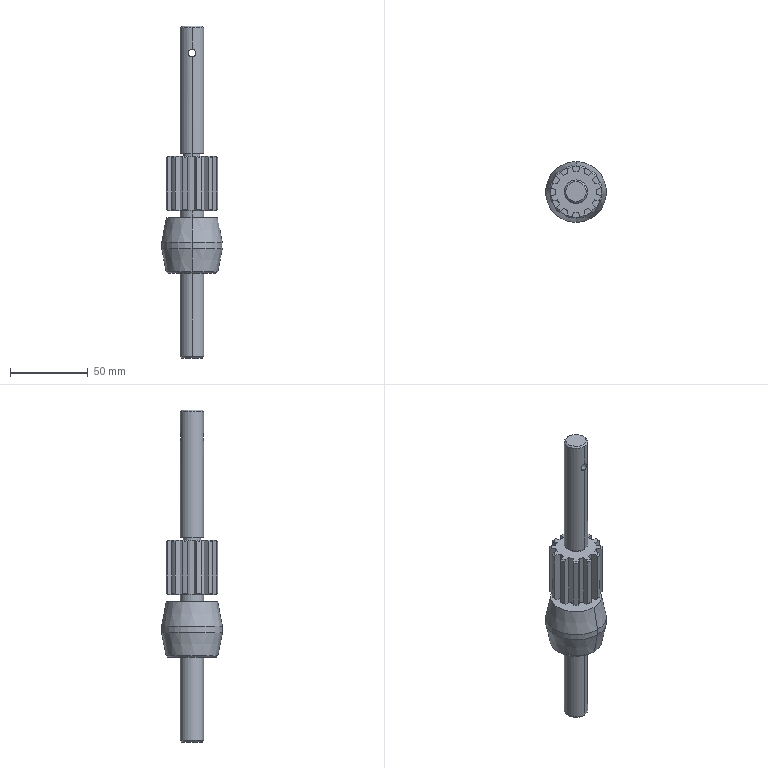Component | SolidWorks | Handwheel-2 | 2 solids | 102 faces | box 39.22 x 39.22 x 214 mm | volume 86786 mm3 | plane 44 | cone 34 | cylinder 24 | commonest cylinder face diameters 34 x12 15 x6 39.22 x2 5 x2 11 x2
build123d program:
from build123d import *
from OCP.BRepFilletAPI import BRepFilletAPI_MakeChamfer

# Parameters (mm, degrees)
SKETCH1_R                = 7.5
BOSS_EXTRUDE1_DEPTH      = 33
SKETCH2_R                = 5.5
BOSS_EXTRUDE2_DEPTH      = 2
SKETCH3_R                = 17
BOSS_EXTRUDE3_DEPTH      = 35
SKETCH4_R                = 7.5
BOSS_EXTRUDE4_DEPTH      = 4.5
SKETCH6_R                = 7.5
BOSS_EXTRUDE5_DEPTH      = 54.5
CHAMFER1_SIZE            = 1
CHAMFER1_SIZE2           = 1.265
CHAMFER2_SIZE            = 1
CHAMFER3_SIZE            = 1
CUT_EXTRUDE1_DEPTH       = 40
CIRPATTERN1_COUNT        = 12
BOSS_EXTRUDE6_DEPTH      = 49
BOSS_EXTRUDE6_DEPTH_BACK = 10
SKETCH8_R                = 7.5
CHAMFER4_SIZE            = 1
CUT_EXTRUDE2_DEPTH       = 168.314
CUT_EXTRUDE2_DEPTH_BACK  = 168.314
SKETCH9_R                = 2.5


with BuildPart() as part:
    # Sketch1 → Boss-Extrude1 (new body)
    with BuildSketch(Plane.XY):
        Circle(SKETCH1_R)
    extrude(amount=BOSS_EXTRUDE1_DEPTH)

    # Sketch2 → Boss-Extrude2 (add)
    with BuildSketch(Plane.XY.offset(33)):
        Circle(SKETCH2_R)
    extrude(amount=BOSS_EXTRUDE2_DEPTH)

    # Sketch3 → Boss-Extrude3 (add)
    with BuildSketch(Plane.XY.offset(35)):
        Circle(SKETCH3_R)
    extrude(amount=BOSS_EXTRUDE3_DEPTH)

    # Sketch4 → Boss-Extrude4 (add)
    with BuildSketch(Plane.XY.offset(70)):
        Circle(SKETCH4_R)
    extrude(amount=BOSS_EXTRUDE4_DEPTH)

    # Chamfer2
    chamfer2_edges = [part.edges().sort_by_distance(p)[0] for p in [
        (-17, 0, 35),
        (-7.5, 0, 0),
    ]]
    chamfer(chamfer2_edges, length=CHAMFER2_SIZE)

    # Chamfer3
    chamfer3_edges = [part.edges().sort_by_distance(p)[0] for p in [
        (-17, 0, 70),
    ]]
    chamfer(chamfer3_edges, length=CHAMFER3_SIZE)

    # Sketch7 → Cut-Extrude1 (cut)
    with BuildSketch(Plane(origin=(0, 0, 35), x_dir=(-1, 0, 0), z_dir=(0, 0, -1))):
        Polygon((-3, 17), (3, 17), (1.456, 13), (-1.544, 13), align=None)
    cut_extrude1 = extrude(amount=-CUT_EXTRUDE1_DEPTH, mode=Mode.SUBTRACT)

    # CirPattern1: Cut-Extrude1 ×12 about axis
    cirpattern1_axis = Axis((0, 0, 0), (0, 0, 1))
    for i in range(1, CIRPATTERN1_COUNT):
        add(cut_extrude1.rotate(cirpattern1_axis, i * 360 / CIRPATTERN1_COUNT), mode=Mode.SUBTRACT)

    # Sketch8 → Boss-Extrude6 (add, two sides: drawn at the far end of the back side and taken through both)
    with BuildSketch(Plane(origin=(0, 0, 0), x_dir=(-1, 0, 0), z_dir=(0, 0, -1)).offset(-BOSS_EXTRUDE6_DEPTH_BACK)):
        with Locations(Location((0, 0, 0), (0, 0, 180))):
            Circle(SKETCH8_R)
    extrude(amount=BOSS_EXTRUDE6_DEPTH + BOSS_EXTRUDE6_DEPTH_BACK)

    # Chamfer4
    chamfer4_edges = [part.edges().sort_by_distance(p)[0] for p in [
        (-7.5, 0, -49),
    ]]
    chamfer(chamfer4_edges, length=CHAMFER4_SIZE)

    # Sketch9 → Cut-Extrude2 (cut, two sides: drawn at the far end of the back side and taken through both)
    with BuildSketch(Plane(origin=(0, 0, 0), x_dir=(0, 0, -1), z_dir=(1, 0, 0)).offset(-CUT_EXTRUDE2_DEPTH_BACK)):
        with Locations((31.5, 0)):
            Circle(SKETCH9_R)
    extrude(amount=CUT_EXTRUDE2_DEPTH + CUT_EXTRUDE2_DEPTH_BACK, mode=Mode.SUBTRACT)


with BuildPart() as body_2:
    # Sketch5 → Revolve1 (revolve)
    with BuildSketch(Plane(origin=(0, 0, 0), x_dir=(1, 0, 0), z_dir=(0, 1, 0))):
        Polygon((0, -74.5), (-16.5, -74.5), (-19.61, -90.5), (-19.61, -94.5), (-16.5, -110.5), (0, -110.5), align=None)
    revolve(axis=Axis((0, 0, 0), (0, 0, 1)))

    # Sketch6 → Boss-Extrude5 (add)
    with BuildSketch(Plane.XY.offset(110.5)):
        Circle(SKETCH6_R)
    extrude(amount=BOSS_EXTRUDE5_DEPTH)

    # Chamfer1: one chamfer whose edges measure the first distance from different faces: ONE call of the kernel's chamfer builder (chamfer() names one face for all edges)
    chamfer1_edges_1 = [body_2.edges().sort_by_distance(p)[0] for p in [
        (-7.5, 0, 165),
    ]]
    chamfer1_edges_2 = [body_2.edges().sort_by_distance(p)[0] for p in [
        (16.5, 0, 110.5),
    ]]
    chamfer1_side_2 = [body_2.faces().sort_by_distance(p)[0] for p in [
        (16.033, 0, 110.5),
    ]]
    chamfer1 = BRepFilletAPI_MakeChamfer(body_2.part.solid().wrapped)
    for e in chamfer1_edges_1:
        chamfer1.Add(CHAMFER1_SIZE, e.wrapped)
    for e in chamfer1_edges_2:
        chamfer1.Add(CHAMFER1_SIZE, CHAMFER1_SIZE2, e.wrapped, chamfer1_side_2[0].wrapped)  # the first distance lies on this face
    add(Compound.cast(chamfer1.Shape()), mode=Mode.REPLACE)


solid = Compound([part.part, body_2.part])

# Placed as in the assembly
solid = solid.moved(Location((32, 58.948, 53), (180, 0, -90)))